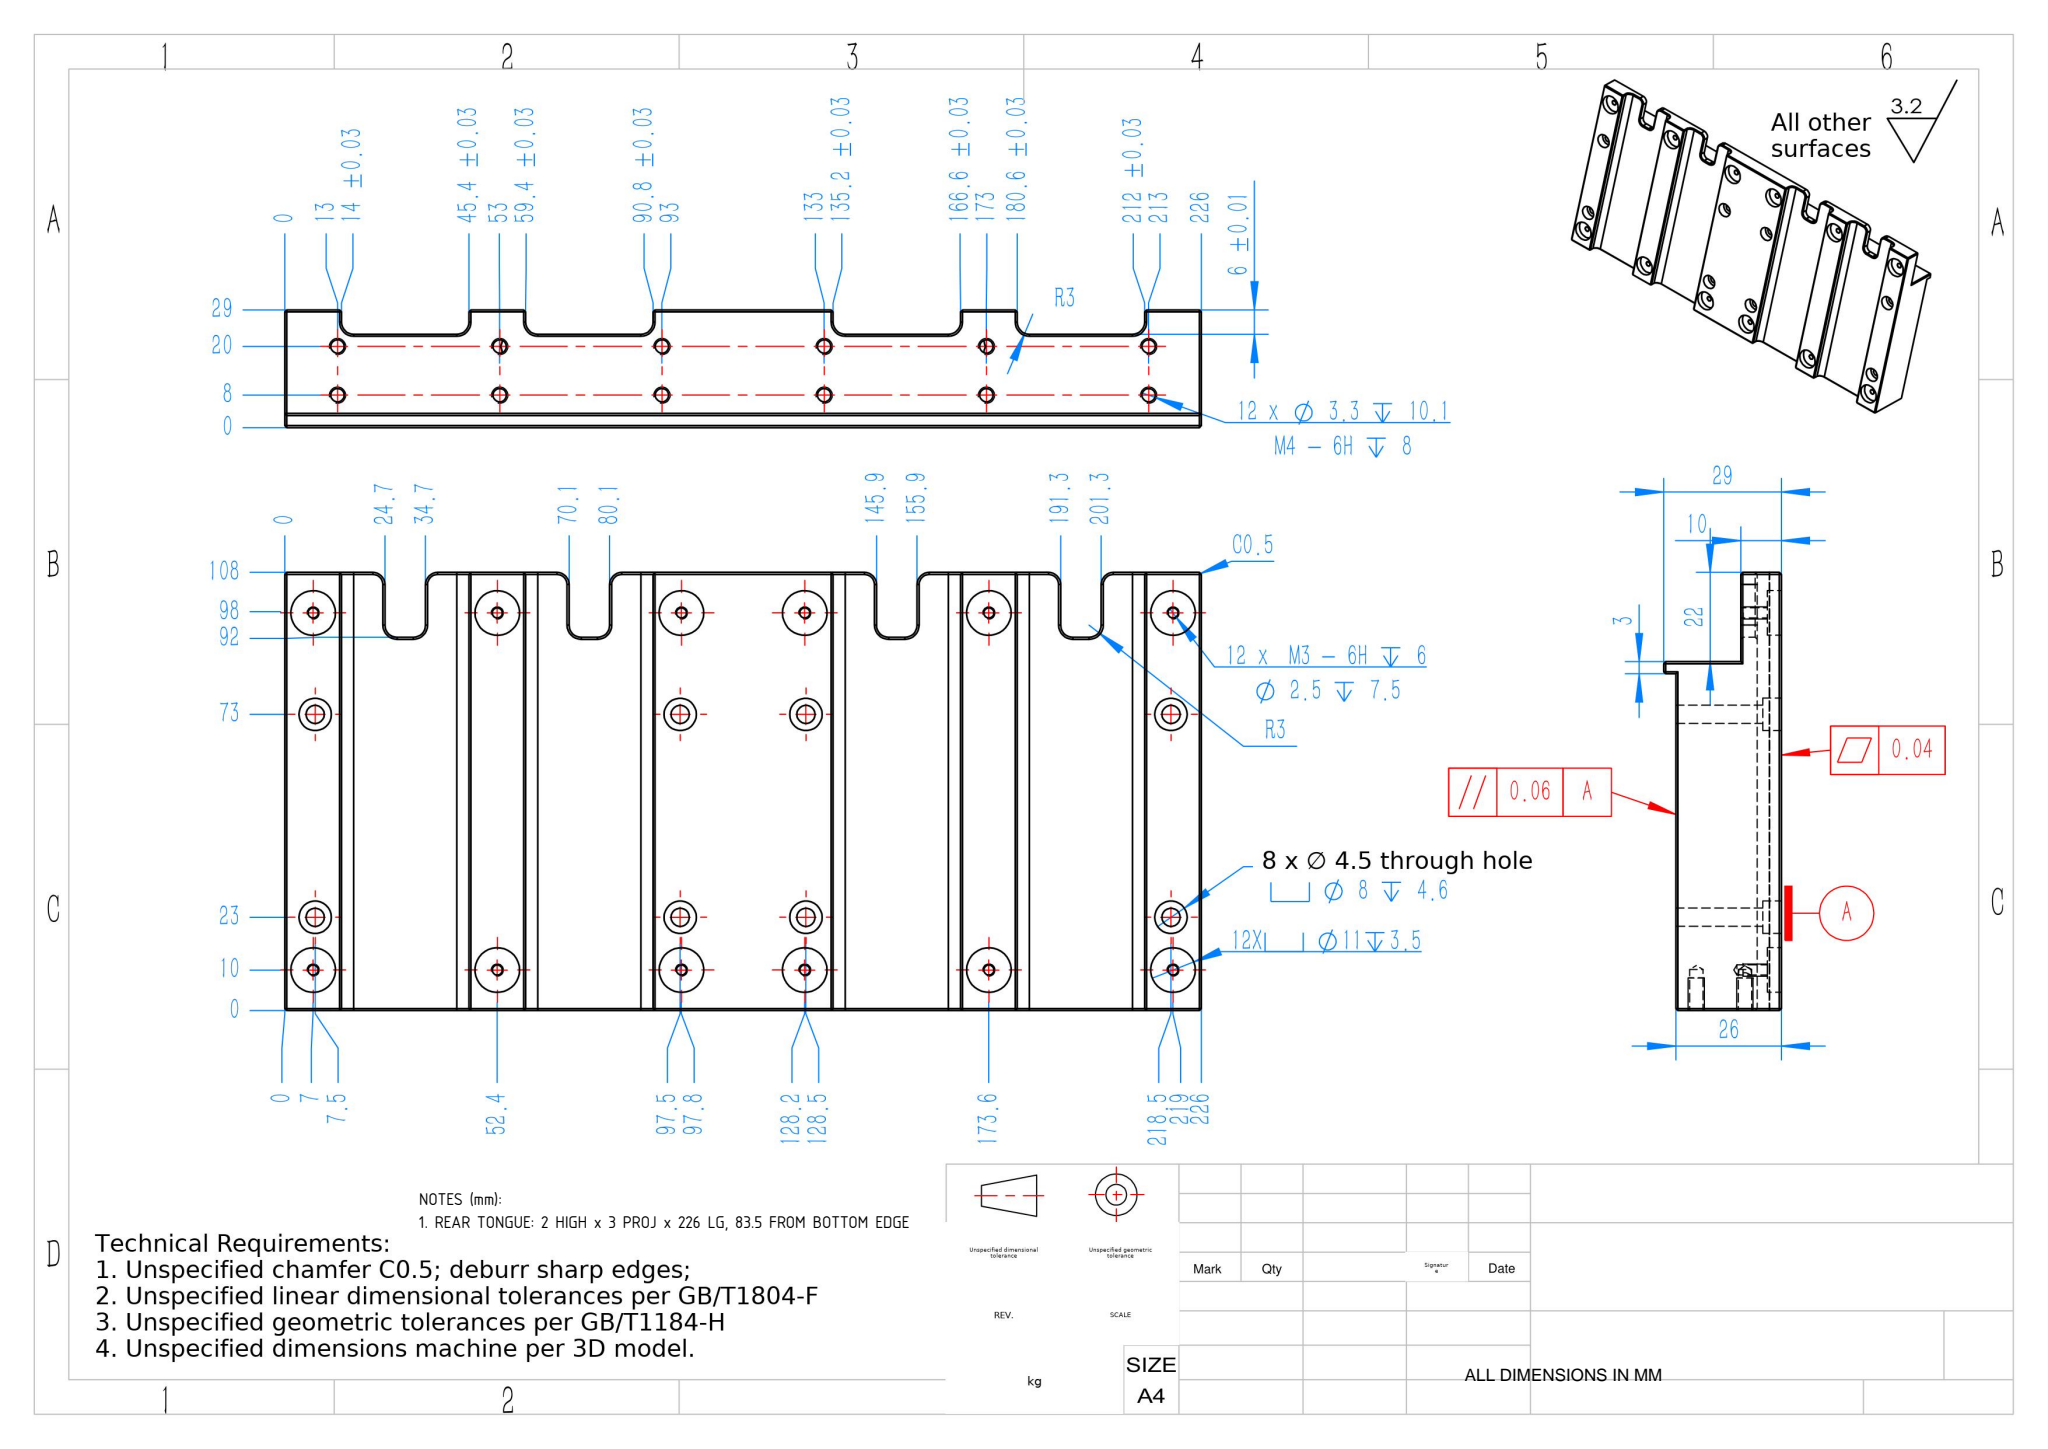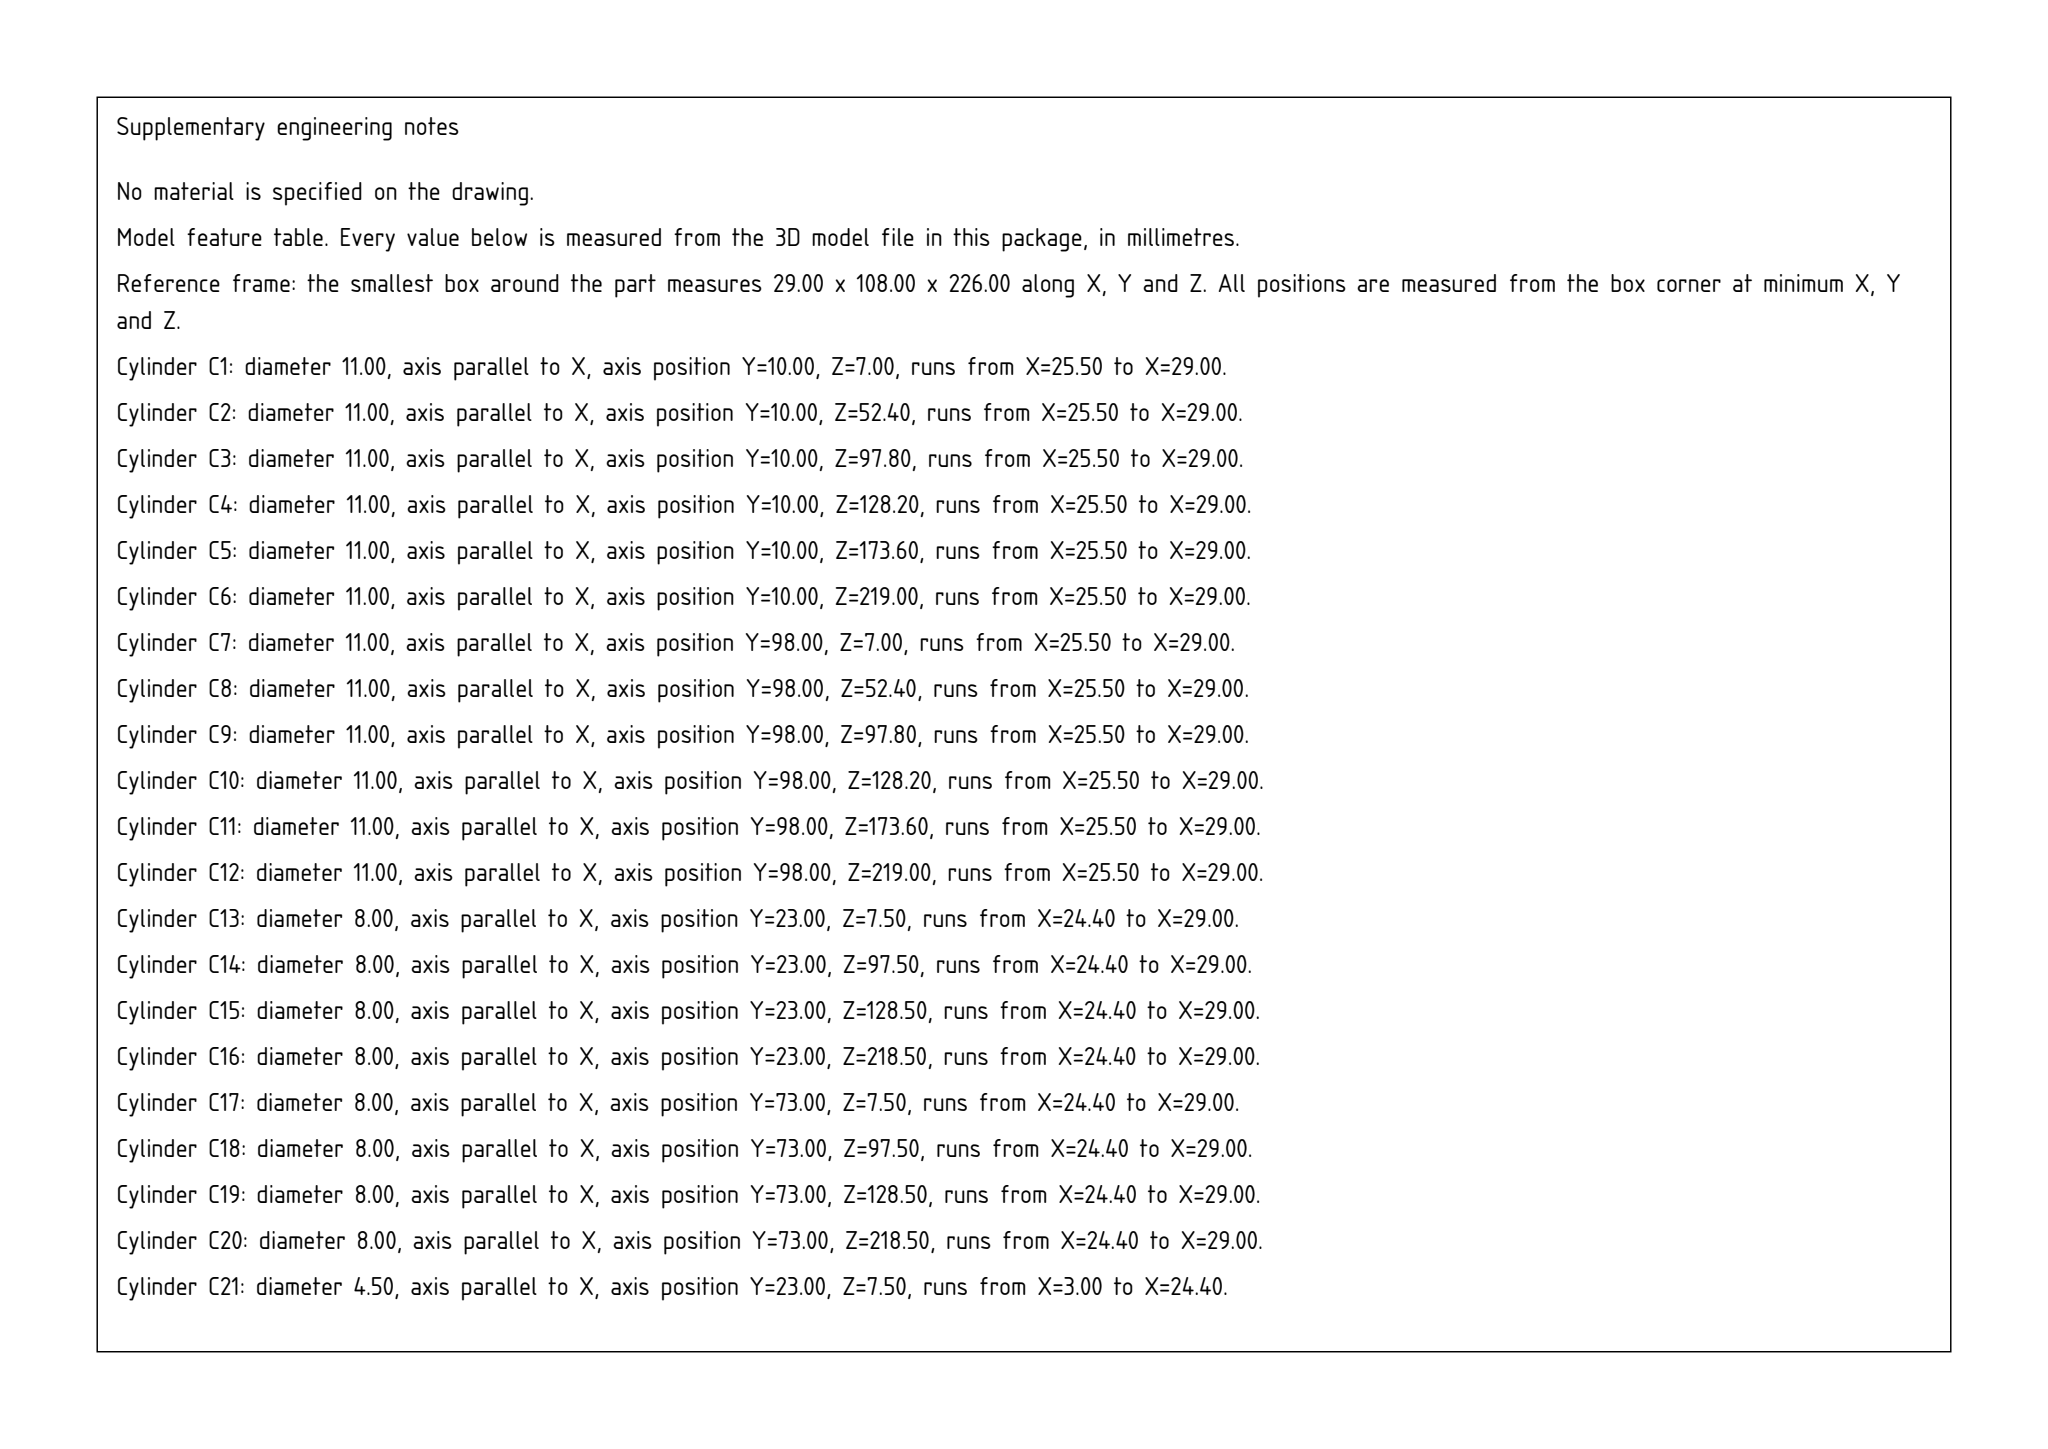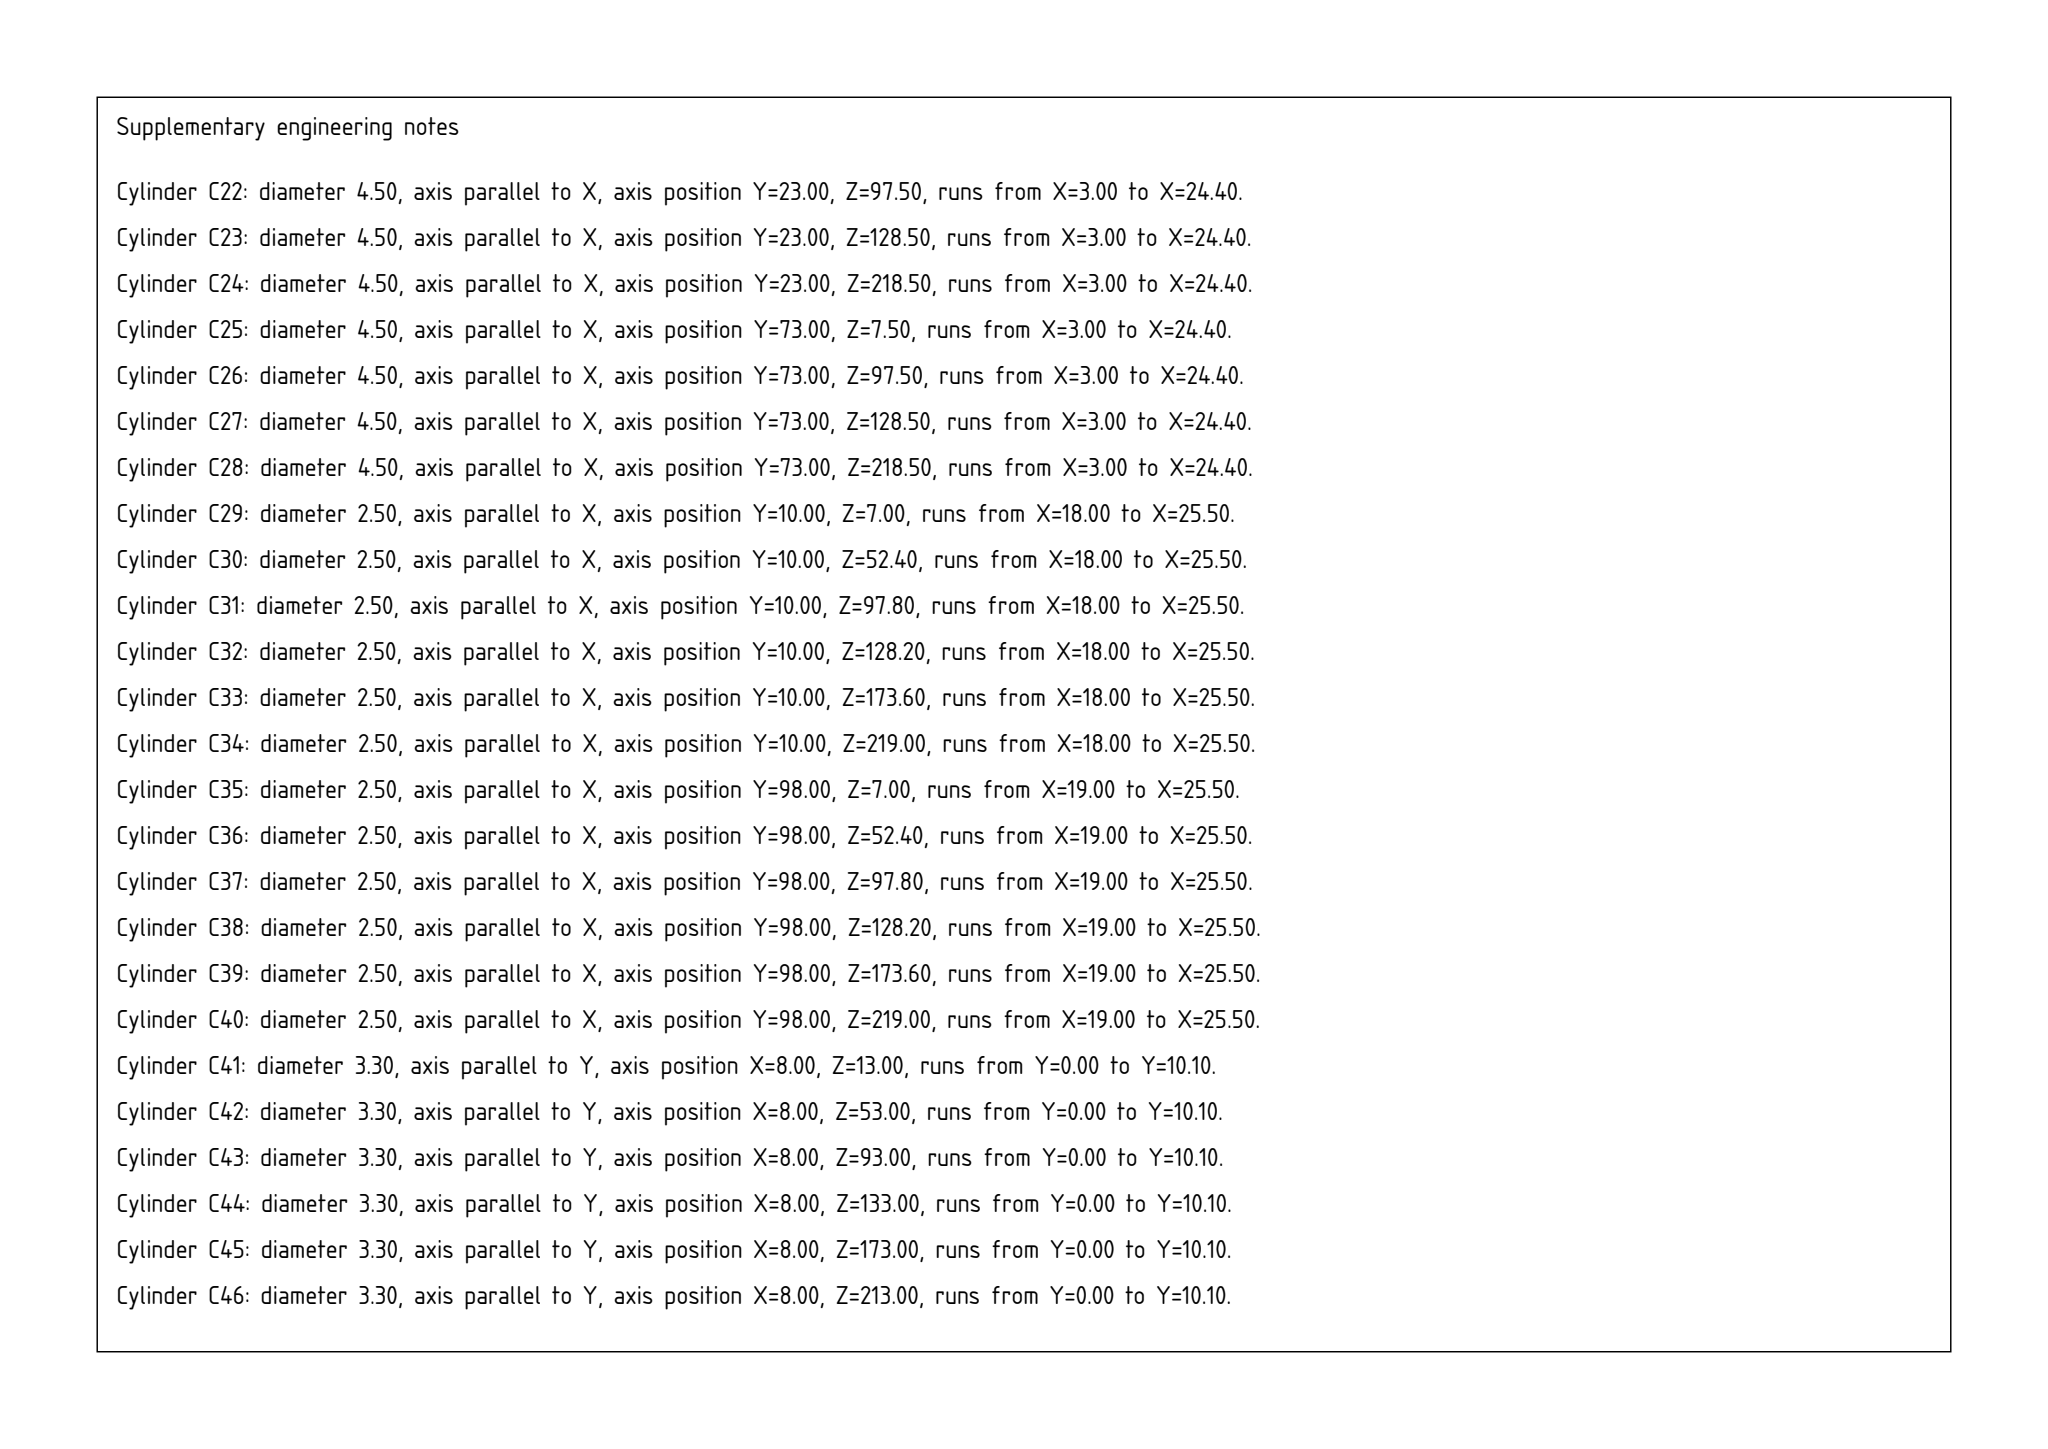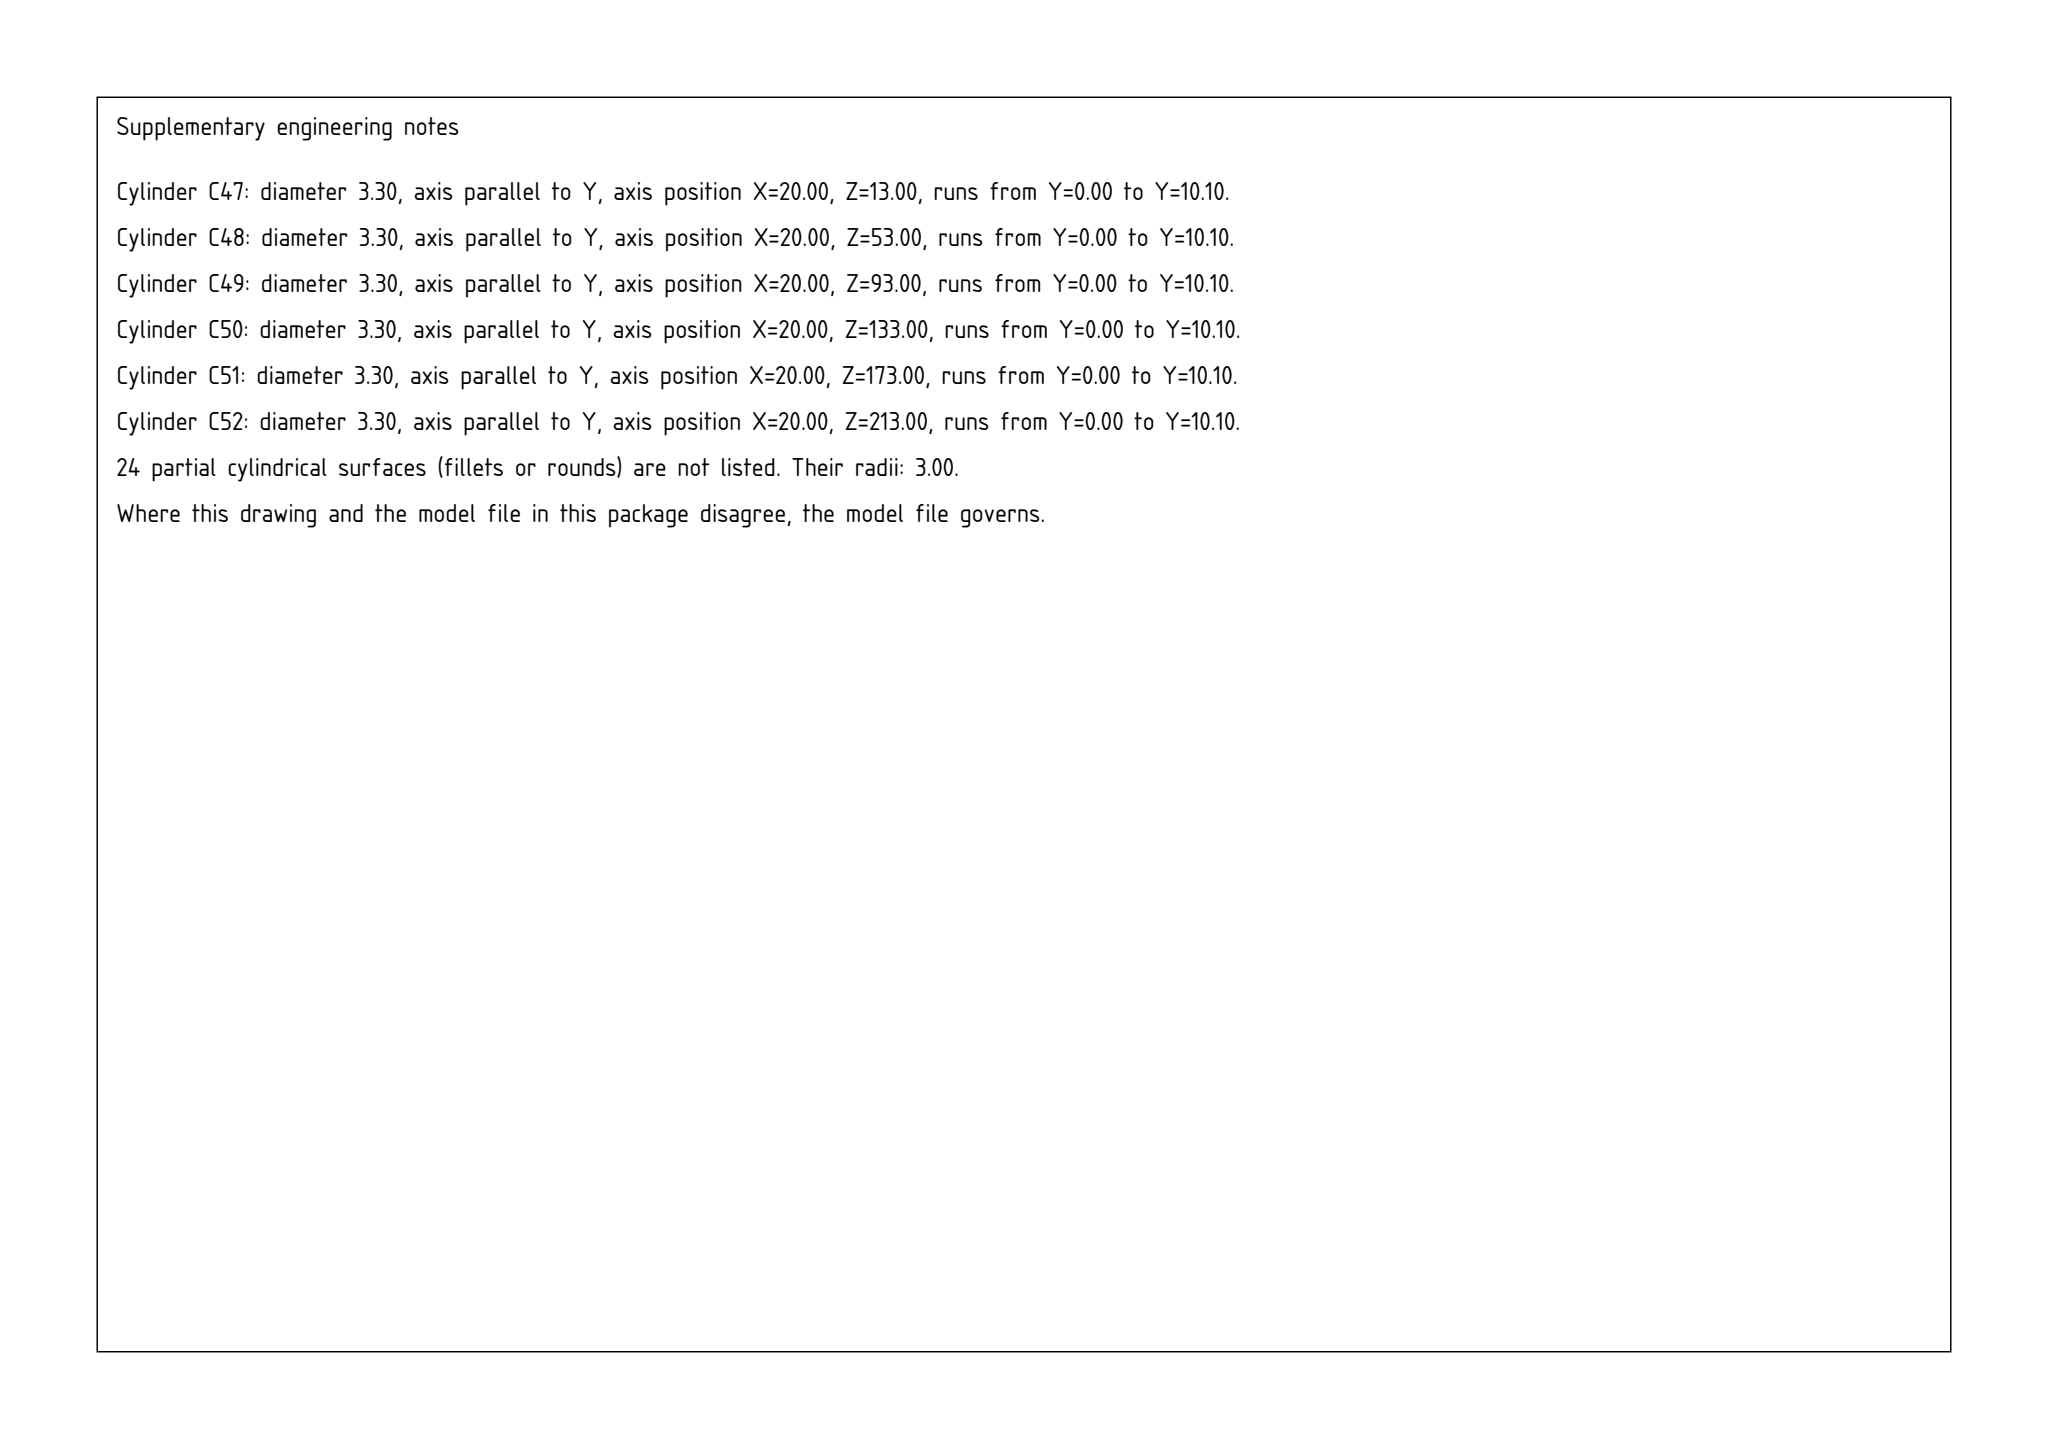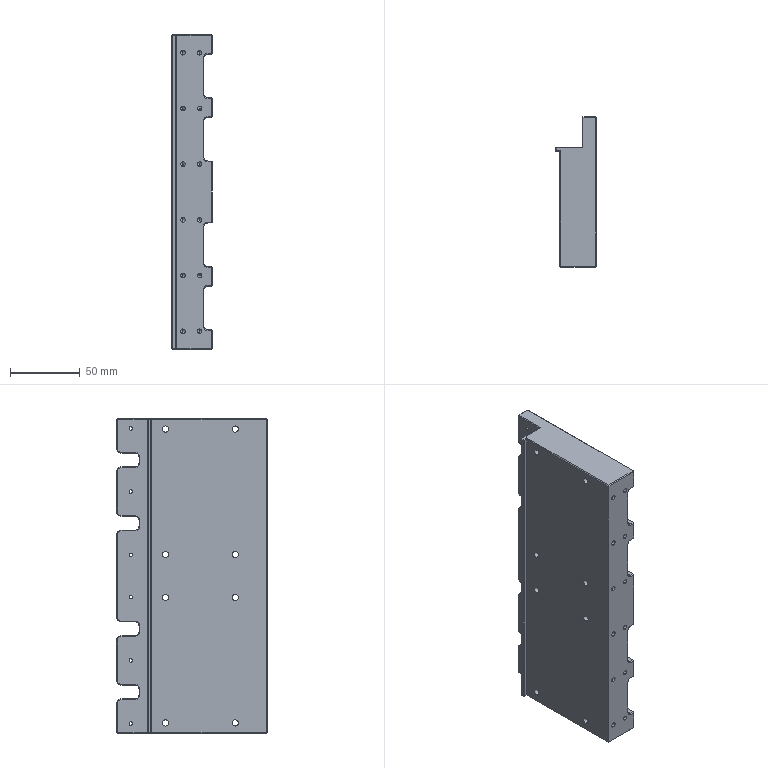Part | SolidWorks | mm | 1 solid | 395 faces | box 29 x 108 x 226 mm | volume 464394 mm3 | plane 184 | cylinder 128 | cone 83 | commonest cylinder face diameters 3.3 x24 2.5 x24 11 x24 6 x24 8 x16 4.5 x16
Drawing notes:
REAR TONGUE: 2 HIGH x 3 PROJ x 226 LG, 83.5 FROM BOTTOM EDGE | from the solid: axis_plane x=0.0, extent y[83.5,85.5] z[0.5,225.5]; back face plane x=3.0 (y 0.5-83.0) => 3 proj, 2 tall, full 226 length; Y from bbox min = drawing 0 datum at bottom edge
build123d program:
from build123d import *

# Parameters (mm, degrees)
SKETCH2_W                                         = 29
SKETCH2_H                                         = 226
BOSS_EXTRUDE1_DEPTH                               = 108
SKETCH3_W                                         = 3
SKETCH3_H                                         = 83
SKETCH3_W_2                                       = 19
SKETCH3_H_2                                       = 22
CUT_EXTRUDE1_DEPTH                                = 251.899
SKETCH4_W                                         = 31.4
SKETCH4_H                                         = 108
CUT_EXTRUDE2_DEPTH                                = 6
HOLE_SIZE_ACCORDING_TO_HEX_SOCKET_HEA_D           = 4.5
HOLE_SIZE_ACCORDING_TO_HEX_SOCKET_HEA_CBORE_D     = 8
HOLE_SIZE_ACCORDING_TO_HEX_SOCKET_HEA_CBORE_DEPTH = 4.6
SKETCH7_W                                         = 10
SKETCH7_H                                         = 32
CUT_EXTRUDE3_DEPTH                                = 158.461
SKETCH8_R                                         = 5.5
CUT_EXTRUDE4_DEPTH                                = 3.5
M3_TAPPED_HOLE1_D                                 = 2.5
M3_TAPPED_HOLE1_DEPTH                             = 7.5
M3_TAPPED_HOLE1_TIP                               = 0.7511
FILLET1_R                                         = 3
FILLET2_R                                         = 3
M4_TAPPED_HOLE1_D                                 = 3.3
M4_TAPPED_HOLE1_DEPTH                             = 10.1
M4_TAPPED_HOLE1_TIP                               = 0.9914
CHAMFER1_SIZE                                     = 0.5


with BuildPart() as part:
    # Sketch2 → Boss-Extrude1 (new body)
    with BuildSketch(Plane(origin=(0, 0, 0), x_dir=(1, 0, 0), z_dir=(0, 1, 0))):
        Rectangle(SKETCH2_W, SKETCH2_H)
    extrude(amount=BOSS_EXTRUDE1_DEPTH)

    # Sketch3 → Cut-Extrude1 (cut, through all)
    with BuildSketch(Plane(origin=(0, 0, -113), x_dir=(-1, 0, 0), z_dir=(0, 0, -1))):
        with Locations((13, 41.5)):
            Rectangle(SKETCH3_W, SKETCH3_H)
        with Locations((5, 97)):
            Rectangle(SKETCH3_W_2, SKETCH3_H_2)
    extrude(amount=-CUT_EXTRUDE1_DEPTH, mode=Mode.SUBTRACT)

    # Sketch4 → Cut-Extrude2 (cut)
    with BuildSketch(Plane(origin=(14.5, 0, 0), x_dir=(0, 0, -1), z_dir=(1, 0, 0))):
        with Locations((83.3, 54)):
            Rectangle(SKETCH4_W, SKETCH4_H)
        with Locations((37.9, 54)):
            Rectangle(SKETCH4_W, SKETCH4_H)
        with Locations((-37.9, 54)):
            Rectangle(SKETCH4_W, SKETCH4_H)
        with Locations((-83.3, 54)):
            Rectangle(SKETCH4_W, SKETCH4_H)
    extrude(amount=-CUT_EXTRUDE2_DEPTH, mode=Mode.SUBTRACT)

    # Hole Size _ according to_ Hex Socket Hea (through all)
    with Locations(Plane(origin=(14.5, 0, 0), x_dir=(0, 0, -1), z_dir=(1, 0, 0))):
        with Locations((-105.5, 73), (-105.5, 23), (-15.5, 23), (-15.5, 73), (15.5, 73), (15.5, 23), (105.5, 23), (105.5, 73)):
            CounterBoreHole(HOLE_SIZE_ACCORDING_TO_HEX_SOCKET_HEA_D / 2, HOLE_SIZE_ACCORDING_TO_HEX_SOCKET_HEA_CBORE_D / 2, HOLE_SIZE_ACCORDING_TO_HEX_SOCKET_HEA_CBORE_DEPTH)

    # Sketch7 → Cut-Extrude3 (cut, through all)
    with BuildSketch(Plane.ZY.offset(-4.5)):
        with Locations((-83.3, 108)):
            Rectangle(SKETCH7_W, SKETCH7_H)
        with Locations((-37.9, 108)):
            Rectangle(SKETCH7_W, SKETCH7_H)
        with Locations((37.9, 108)):
            Rectangle(SKETCH7_W, SKETCH7_H)
        with Locations((83.3, 108)):
            Rectangle(SKETCH7_W, SKETCH7_H)
    extrude(amount=-CUT_EXTRUDE3_DEPTH, mode=Mode.SUBTRACT)

    # Sketch8 → Cut-Extrude4 (cut)
    with BuildSketch(Plane(origin=(14.5, 0, 0), x_dir=(0, 0, -1), z_dir=(1, 0, 0))):
        with Locations((-106, 98)):
            Circle(SKETCH8_R)
        with Locations(Location((-106, 10, 0), (0, 0, 180))):
            Circle(SKETCH8_R)
        with Locations((-60.6, 10)):
            Circle(SKETCH8_R)
        with Locations(Location((-60.6, 98, 0), (0, 0, 180))):
            Circle(SKETCH8_R)
        with Locations((-15.2, 98)):
            Circle(SKETCH8_R)
        with Locations(Location((-15.2, 10, 0), (0, 0, 180))):
            Circle(SKETCH8_R)
        with Locations((15.2, 10)):
            Circle(SKETCH8_R)
        with Locations(Location((15.2, 98, 0), (0, 0, 180))):
            Circle(SKETCH8_R)
        with Locations((60.6, 98)):
            Circle(SKETCH8_R)
        with Locations(Location((60.6, 10, 0), (0, 0, 180))):
            Circle(SKETCH8_R)
        with Locations((106, 10)):
            Circle(SKETCH8_R)
        with Locations(Location((106, 98, 0), (0, 0, 180))):
            Circle(SKETCH8_R)
    extrude(amount=-CUT_EXTRUDE4_DEPTH, mode=Mode.SUBTRACT)

    # M3 Tapped Hole1
    with Locations(Plane(origin=(11, 0, 0), x_dir=(0, 0, -1), z_dir=(1, 0, 0))):
        with Locations((-106, 98), (-106, 10), (-60.6, 98), (-60.6, 10), (-15.2, 98), (15.2, 98), (60.6, 98), (106, 98), (106, 10), (60.6, 10), (15.2, 10), (-15.2, 10)):
            Hole(M3_TAPPED_HOLE1_D / 2, depth=M3_TAPPED_HOLE1_DEPTH)
            with Locations((0, 0, -(M3_TAPPED_HOLE1_DEPTH + M3_TAPPED_HOLE1_TIP / 2))):  # 118° drill point
                Cone(0, M3_TAPPED_HOLE1_D / 2, M3_TAPPED_HOLE1_TIP, mode=Mode.SUBTRACT)

    # Fillet1
    fillet1_edges = [part.edges().sort_by_distance(p)[0] for p in [
        (6.5, 108, -88.3),
        (6.5, 108, -78.3),
        (6.5, 92, -78.3),
        (6.5, 92, -88.3),
        (6.5, 108, -42.9),
        (6.5, 108, -32.9),
        (6.5, 92, -42.9),
        (6.5, 92, -32.9),
        (6.5, 108, 42.9),
        (6.5, 92, 42.9),
        (6.5, 108, 32.9),
        (6.5, 92, 32.9),
        (6.5, 108, 78.3),
        (6.5, 108, 88.3),
        (6.5, 92, 78.3),
        (6.5, 92, 88.3),
    ]]
    fillet(fillet1_edges, radius=FILLET1_R)

    # Fillet2
    fillet2_edges = [part.edges().sort_by_distance(p)[0] for p in [
        (8.5, 54, -99),
        (8.5, 54, -67.6),
        (8.5, 54, -53.6),
        (8.5, 54, -22.2),
        (8.5, 54, 53.6),
        (8.5, 54, 22.2),
        (8.5, 54, 67.6),
        (8.5, 54, 99),
    ]]
    fillet(fillet2_edges, radius=FILLET2_R)

    # M4 Tapped Hole1
    with Locations(Plane(origin=(0, 0, 0), x_dir=(-1, 0, 0), z_dir=(0, -1, 0))):
        with Locations((6.5, 100), (-5.5, 100), (6.5, 60), (-5.5, 60), (6.5, 20), (-5.5, 20), (6.5, -20), (-5.5, -20), (6.5, -60), (-5.5, -60), (6.5, -100), (-5.5, -100)):
            Hole(M4_TAPPED_HOLE1_D / 2, depth=M4_TAPPED_HOLE1_DEPTH)
            with Locations((0, 0, -(M4_TAPPED_HOLE1_DEPTH + M4_TAPPED_HOLE1_TIP / 2))):  # 118° drill point
                Cone(0, M4_TAPPED_HOLE1_D / 2, M4_TAPPED_HOLE1_TIP, mode=Mode.SUBTRACT)

    # Chamfer1
    chamfer1_edges = [part.edges().sort_by_distance(p)[0] for p in [
        (1.5, 0, 113),
        (9.5, 108, 113),
        (-14.5, 84.5, 113),
        (-14.5, 84.5, -113),
        (-14.5, 83, 0),
        (-11.5, 41.5, 113),
        (-11.5, 0, 0),
        (-13, 83, 113),
        (-13, 83, -113),
        (-11.5, 41.5, -113),
        (-5, 86, 113),
        (-14.5, 86, 0),
        (4.5, 97, 113),
        (4.5, 108, 102.15),
        (4.5, 97, -113),
        (-5, 86, -113),
        (4.5, 92, -83.3),
        (8.5, 92, -83.3),
        (4.5, 100, -88.3),
        (8.5, 100, -88.3),
        (8.5, 100, -78.3),
        (4.5, 100, -78.3),
        (4.5, 108, -102.15),
        (4.5, 100, 88.3),
        (4.5, 92, 83.3),
        (4.5, 100, 78.3),
        (4.5, 108, 60.6),
        (4.5, 100, 42.9),
        (4.5, 92, 37.9),
        (4.5, 100, 32.9),
        (4.5, 108, 0),
        (4.5, 100, -32.9),
        (4.5, 92, -37.9),
        (4.5, 100, -42.9),
        (4.5, 108, -60.6),
        (4.5, 107.121, 89.179),
        (4.5, 107.121, 77.421),
        (4.5, 107.121, 32.021),
        (4.5, 107.121, 43.779),
        (4.5, 107.121, -32.021),
        (4.5, 107.121, -43.779),
        (4.5, 107.121, -77.421),
        (4.5, 107.121, -89.179),
        (8.5, 108, -72.95),
        (8.5, 107.121, -77.421),
        (8.5, 107.121, -89.179),
        (8.5, 92, -37.9),
        (8.5, 100, -42.9),
        (8.5, 100, -32.9),
        (8.5, 108, -27.55),
        (8.5, 107.121, -32.021),
        (8.5, 107.121, -43.779),
        (8.5, 92, 37.9),
        (8.5, 100, 32.9),
        (8.5, 100, 42.9),
        (8.5, 108, 48.25),
        (8.5, 107.121, 32.021),
        (8.5, 107.121, 43.779),
        (8.5, 100, 78.3),
        (8.5, 92, 83.3),
        (8.5, 100, 88.3),
        (8.5, 108, 93.65),
        (8.5, 107.121, 89.179),
        (8.5, 107.121, 77.421),
        (4.5, 92.879, -87.421),
        (8.5, 92.879, -87.421),
        (4.5, 92.879, -79.179),
        (8.5, 92.879, -79.179),
        (4.5, 92.879, -42.021),
        (8.5, 92.879, -42.021),
        (4.5, 92.879, -33.779),
        (8.5, 92.879, -33.779),
        (4.5, 92.879, 33.779),
        (8.5, 92.879, 33.779),
        (4.5, 92.879, 42.021),
        (8.5, 92.879, 42.021),
        (4.5, 92.879, 87.421),
        (8.5, 92.879, 87.421),
        (4.5, 92.879, 79.179),
        (8.5, 92.879, 79.179),
        (14.5, 0, 60.6),
        (14.5, 0, 0),
        (14.5, 0, -60.6),
        (14.5, 0, -106),
        (8.5, 108, -93.65),
        (8.5, 0, -83.3),
        (13, 108, -99),
        (13, 0, -99),
        (13, 0, -67.6),
        (13, 108, -67.6),
        (8.5, 108, -48.25),
        (8.5, 0, -37.9),
        (13, 0, -22.2),
        (13, 108, -22.2),
        (13, 108, -53.6),
        (13, 0, -53.6),
        (8.5, 0, 37.9),
        (8.5, 108, 27.55),
        (13, 108, 22.2),
        (13, 0, 22.2),
        (13, 0, 53.6),
        (13, 108, 53.6),
        (8.5, 108, 72.95),
        (8.5, 0, 83.3),
        (13, 0, 99),
        (13, 108, 99),
        (13, 108, 67.6),
        (13, 0, 67.6),
        (9.379, 108, -98.121),
        (9.379, 0, -98.121),
        (9.379, 0, -68.479),
        (9.379, 108, -68.479),
        (9.379, 0, -23.079),
        (9.379, 108, -23.079),
        (9.379, 108, -52.721),
        (9.379, 0, -52.721),
        (9.379, 108, 23.079),
        (9.379, 0, 23.079),
        (9.379, 0, 52.721),
        (9.379, 108, 52.721),
        (9.379, 0, 98.121),
        (9.379, 108, 98.121),
        (9.379, 108, 68.479),
        (9.379, 0, 68.479),
        (14.5, 108, 106),
        (14.5, 108, 60.6),
        (14.5, 108, 0),
        (14.5, 108, -60.6),
        (14.5, 108, -106),
        (1.5, 0, -113),
        (14.5, 0, 106),
        (14.5, 54, -99),
        (14.5, 54, -67.6),
        (14.5, 54, -53.6),
        (14.5, 54, -22.2),
        (14.5, 54, 53.6),
        (14.5, 54, 22.2),
        (14.5, 54, 113),
        (14.5, 54, 67.6),
        (14.5, 54, 99),
        (14.5, 54, -113),
        (9.5, 108, -113),
    ]]
    chamfer(chamfer1_edges, length=CHAMFER1_SIZE)


solid = part.part